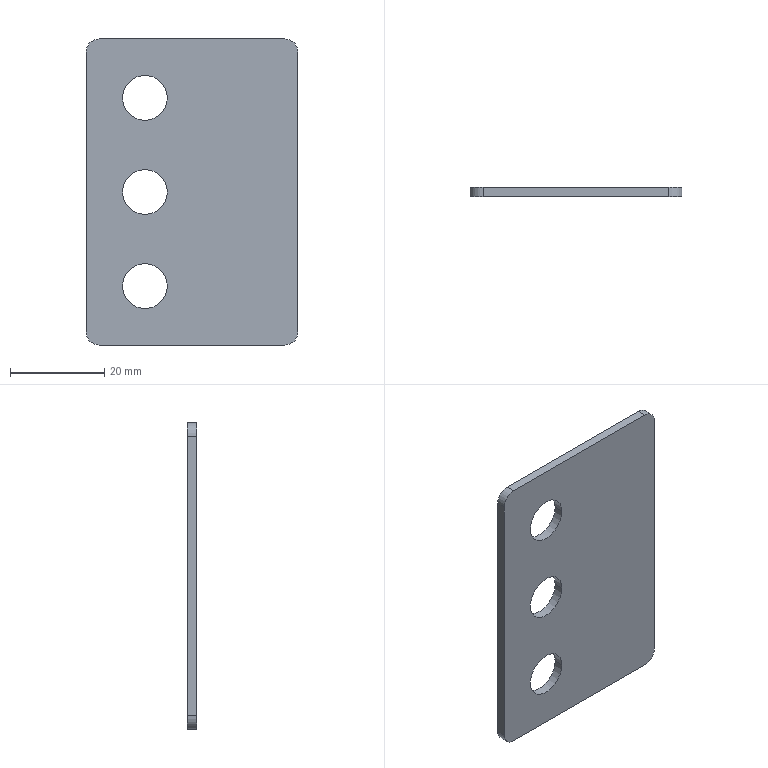Component | SolidWorks | HighVoltageMountingPlateAssembly-1_HighVoltageOutletCabinetMountingPlateSideBaffles-1 | 1 solid | 16 faces | box 45 x 2 x 65 mm | volume 5411 mm3 | cylinder 10 | plane 6 | commonest cylinder face diameters 9.5 x6 5.6 x4 | material Plain Carbon Steel
STEP:
#1=COLOUR_RGB('',0.7922,0.8196,0.9333);
#2=FILL_AREA_STYLE_COLOUR('',#1);
#3=FILL_AREA_STYLE('',(#2));
#4=SURFACE_STYLE_FILL_AREA(#3);
#5=SURFACE_SIDE_STYLE('',(#4));
#6=SURFACE_STYLE_USAGE(.BOTH.,#5);
#7=PRESENTATION_STYLE_ASSIGNMENT((#6));
#8=CARTESIAN_POINT('',(-68.137,3.52,85.837));
#9=VERTEX_POINT('',#8);
#10=CARTESIAN_POINT('',(-68.511,3.52,85.837));
#11=VERTEX_POINT('',#10);
#12=CARTESIAN_POINT('',(-68.324,3.52,85.837));
#13=DIRECTION('',(-0.,1.,-0.));
#14=DIRECTION('',(-1.,0.,0.));
#15=AXIS2_PLACEMENT_3D('',#12,#13,#14);
#16=CIRCLE('',#15,0.187);
#17=EDGE_CURVE('',#9,#11,#16,.T.);
#18=ORIENTED_EDGE('',*,*,#17,.F.);
#19=CARTESIAN_POINT('',(-68.137,3.599,85.837));
#20=VERTEX_POINT('',#19);
#21=CARTESIAN_POINT('',(-68.137,3.52,85.837));
#22=DIRECTION('',(-0.,1.,-0.));
#23=VECTOR('',#22,39.37);
#24=LINE('',#21,#23);
#25=EDGE_CURVE('',#9,#20,#24,.T.);
#26=ORIENTED_EDGE('',*,*,#25,.T.);
#27=CARTESIAN_POINT('',(-68.511,3.599,85.837));
#28=VERTEX_POINT('',#27);
#29=CARTESIAN_POINT('',(-68.324,3.599,85.837));
#30=DIRECTION('',(-0.,1.,-0.));
#31=DIRECTION('',(-1.,0.,0.));
#32=AXIS2_PLACEMENT_3D('',#29,#30,#31);
#33=CIRCLE('',#32,0.187);
#34=EDGE_CURVE('',#20,#28,#33,.T.);
#35=ORIENTED_EDGE('',*,*,#34,.T.);
#36=CARTESIAN_POINT('',(-68.511,3.52,85.837));
#37=DIRECTION('',(-0.,1.,-0.));
#38=VECTOR('',#37,39.37);
#39=LINE('',#36,#38);
#40=EDGE_CURVE('',#11,#28,#39,.T.);
#41=ORIENTED_EDGE('',*,*,#40,.F.);
#42=EDGE_LOOP('',(#18,#26,#35,#41));
#43=FACE_OUTER_BOUND('',#42,.T.);
#44=CARTESIAN_POINT('',(-68.324,3.52,85.837));
#45=DIRECTION('',(-0.,1.,-0.));
#46=DIRECTION('',(-1.,0.,0.));
#47=AXIS2_PLACEMENT_3D('',#44,#45,#46);
#48=CYLINDRICAL_SURFACE('',#47,0.187);
#49=ADVANCED_FACE('',(#43),#48,.F.);
#50=CARTESIAN_POINT('',(-68.137,3.52,85.05));
#51=VERTEX_POINT('',#50);
#52=CARTESIAN_POINT('',(-68.511,3.52,85.05));
#53=VERTEX_POINT('',#52);
#54=CARTESIAN_POINT('',(-68.324,3.52,85.05));
#55=DIRECTION('',(-0.,1.,-0.));
#56=DIRECTION('',(-1.,0.,0.));
#57=AXIS2_PLACEMENT_3D('',#54,#55,#56);
#58=CIRCLE('',#57,0.187);
#59=EDGE_CURVE('',#51,#53,#58,.T.);
#60=ORIENTED_EDGE('',*,*,#59,.F.);
#61=CARTESIAN_POINT('',(-68.137,3.599,85.05));
#62=VERTEX_POINT('',#61);
#63=CARTESIAN_POINT('',(-68.137,3.52,85.05));
#64=DIRECTION('',(-0.,1.,-0.));
#65=VECTOR('',#64,39.37);
#66=LINE('',#63,#65);
#67=EDGE_CURVE('',#51,#62,#66,.T.);
#68=ORIENTED_EDGE('',*,*,#67,.T.);
#69=CARTESIAN_POINT('',(-68.511,3.599,85.05));
#70=VERTEX_POINT('',#69);
#71=CARTESIAN_POINT('',(-68.324,3.599,85.05));
#72=DIRECTION('',(-0.,1.,-0.));
#73=DIRECTION('',(-1.,0.,0.));
#74=AXIS2_PLACEMENT_3D('',#71,#72,#73);
#75=CIRCLE('',#74,0.187);
#76=EDGE_CURVE('',#62,#70,#75,.T.);
#77=ORIENTED_EDGE('',*,*,#76,.T.);
#78=CARTESIAN_POINT('',(-68.511,3.52,85.05));
#79=DIRECTION('',(-0.,1.,-0.));
#80=VECTOR('',#79,39.37);
#81=LINE('',#78,#80);
#82=EDGE_CURVE('',#53,#70,#81,.T.);
#83=ORIENTED_EDGE('',*,*,#82,.F.);
#84=EDGE_LOOP('',(#60,#68,#77,#83));
#85=FACE_OUTER_BOUND('',#84,.T.);
#86=CARTESIAN_POINT('',(-68.324,3.52,85.05));
#87=DIRECTION('',(-0.,1.,-0.));
#88=DIRECTION('',(-1.,0.,0.));
#89=AXIS2_PLACEMENT_3D('',#86,#87,#88);
#90=CYLINDRICAL_SURFACE('',#89,0.187);
#91=ADVANCED_FACE('',(#85),#90,.F.);
#92=CARTESIAN_POINT('',(-68.137,3.52,86.625));
#93=VERTEX_POINT('',#92);
#94=CARTESIAN_POINT('',(-68.511,3.52,86.625));
#95=VERTEX_POINT('',#94);
#96=CARTESIAN_POINT('',(-68.324,3.52,86.625));
#97=DIRECTION('',(-0.,1.,-0.));
#98=DIRECTION('',(-1.,0.,0.));
#99=AXIS2_PLACEMENT_3D('',#96,#97,#98);
#100=CIRCLE('',#99,0.187);
#101=EDGE_CURVE('',#93,#95,#100,.T.);
#102=ORIENTED_EDGE('',*,*,#101,.F.);
#103=CARTESIAN_POINT('',(-68.137,3.599,86.625));
#104=VERTEX_POINT('',#103);
#105=CARTESIAN_POINT('',(-68.137,3.52,86.625));
#106=DIRECTION('',(-0.,1.,-0.));
#107=VECTOR('',#106,39.37);
#108=LINE('',#105,#107);
#109=EDGE_CURVE('',#93,#104,#108,.T.);
#110=ORIENTED_EDGE('',*,*,#109,.T.);
#111=CARTESIAN_POINT('',(-68.511,3.599,86.625));
#112=VERTEX_POINT('',#111);
#113=CARTESIAN_POINT('',(-68.324,3.599,86.625));
#114=DIRECTION('',(-0.,1.,-0.));
#115=DIRECTION('',(-1.,0.,0.));
#116=AXIS2_PLACEMENT_3D('',#113,#114,#115);
#117=CIRCLE('',#116,0.187);
#118=EDGE_CURVE('',#104,#112,#117,.T.);
#119=ORIENTED_EDGE('',*,*,#118,.T.);
#120=CARTESIAN_POINT('',(-68.511,3.52,86.625));
#121=DIRECTION('',(-0.,1.,-0.));
#122=VECTOR('',#121,39.37);
#123=LINE('',#120,#122);
#124=EDGE_CURVE('',#95,#112,#123,.T.);
#125=ORIENTED_EDGE('',*,*,#124,.F.);
#126=EDGE_LOOP('',(#102,#110,#119,#125));
#127=FACE_OUTER_BOUND('',#126,.T.);
#128=CARTESIAN_POINT('',(-68.324,3.52,86.625));
#129=DIRECTION('',(-0.,1.,-0.));
#130=DIRECTION('',(-1.,0.,0.));
#131=AXIS2_PLACEMENT_3D('',#128,#129,#130);
#132=CYLINDRICAL_SURFACE('',#131,0.187);
#133=ADVANCED_FACE('',(#127),#132,.F.);
#134=CARTESIAN_POINT('',(-67.045,3.52,87.007));
#135=VERTEX_POINT('',#134);
#136=CARTESIAN_POINT('',(-67.045,3.52,84.668));
#137=VERTEX_POINT('',#136);
#138=CARTESIAN_POINT('',(-67.045,3.52,84.558));
#139=DIRECTION('',(-0.,0.,-1.));
#140=VECTOR('',#139,39.37);
#141=LINE('',#138,#140);
#142=EDGE_CURVE('',#135,#137,#141,.T.);
#143=ORIENTED_EDGE('',*,*,#142,.T.);
#144=CARTESIAN_POINT('',(-67.045,3.599,84.668));
#145=VERTEX_POINT('',#144);
#146=CARTESIAN_POINT('',(-67.045,3.52,84.668));
#147=DIRECTION('',(-0.,1.,-0.));
#148=VECTOR('',#147,39.37);
#149=LINE('',#146,#148);
#150=EDGE_CURVE('',#137,#145,#149,.T.);
#151=ORIENTED_EDGE('',*,*,#150,.T.);
#152=CARTESIAN_POINT('',(-67.045,3.599,87.007));
#153=VERTEX_POINT('',#152);
#154=CARTESIAN_POINT('',(-67.045,3.599,84.558));
#155=DIRECTION('',(-0.,0.,-1.));
#156=VECTOR('',#155,39.37);
#157=LINE('',#154,#156);
#158=EDGE_CURVE('',#153,#145,#157,.T.);
#159=ORIENTED_EDGE('',*,*,#158,.F.);
#160=CARTESIAN_POINT('',(-67.045,3.52,87.007));
#161=DIRECTION('',(0.,-1.,0.));
#162=VECTOR('',#161,39.37);
#163=LINE('',#160,#162);
#164=EDGE_CURVE('',#153,#135,#163,.T.);
#165=ORIENTED_EDGE('',*,*,#164,.T.);
#166=EDGE_LOOP('',(#143,#151,#159,#165));
#167=FACE_OUTER_BOUND('',#166,.T.);
#168=CARTESIAN_POINT('',(-67.045,3.52,84.558));
#169=DIRECTION('',(1.,0.,0.));
#170=DIRECTION('',(-0.,1.,-0.));
#171=AXIS2_PLACEMENT_3D('',#168,#169,#170);
#172=PLANE('',#171);
#173=ADVANCED_FACE('',(#167),#172,.T.);
#174=CARTESIAN_POINT('',(-68.706,3.599,87.117));
#175=VERTEX_POINT('',#174);
#176=CARTESIAN_POINT('',(-67.155,3.599,87.117));
#177=VERTEX_POINT('',#176);
#178=CARTESIAN_POINT('',(-67.045,3.599,87.117));
#179=DIRECTION('',(1.,-0.,0.));
#180=VECTOR('',#179,39.37);
#181=LINE('',#178,#180);
#182=EDGE_CURVE('',#175,#177,#181,.T.);
#183=ORIENTED_EDGE('',*,*,#182,.F.);
#184=CARTESIAN_POINT('',(-68.706,3.52,87.117));
#185=VERTEX_POINT('',#184);
#186=CARTESIAN_POINT('',(-68.706,3.52,87.117));
#187=DIRECTION('',(0.,-1.,0.));
#188=VECTOR('',#187,39.37);
#189=LINE('',#186,#188);
#190=EDGE_CURVE('',#175,#185,#189,.T.);
#191=ORIENTED_EDGE('',*,*,#190,.T.);
#192=CARTESIAN_POINT('',(-67.155,3.52,87.117));
#193=VERTEX_POINT('',#192);
#194=CARTESIAN_POINT('',(-67.045,3.52,87.117));
#195=DIRECTION('',(1.,-0.,0.));
#196=VECTOR('',#195,39.37);
#197=LINE('',#194,#196);
#198=EDGE_CURVE('',#185,#193,#197,.T.);
#199=ORIENTED_EDGE('',*,*,#198,.T.);
#200=CARTESIAN_POINT('',(-67.155,3.52,87.117));
#201=DIRECTION('',(-0.,1.,-0.));
#202=VECTOR('',#201,39.37);
#203=LINE('',#200,#202);
#204=EDGE_CURVE('',#193,#177,#203,.T.);
#205=ORIENTED_EDGE('',*,*,#204,.T.);
#206=EDGE_LOOP('',(#183,#191,#199,#205));
#207=FACE_OUTER_BOUND('',#206,.T.);
#208=CARTESIAN_POINT('',(-67.045,3.52,87.117));
#209=DIRECTION('',(0.,0.,1.));
#210=DIRECTION('',(-0.,1.,-0.));
#211=AXIS2_PLACEMENT_3D('',#208,#209,#210);
#212=PLANE('',#211);
#213=ADVANCED_FACE('',(#207),#212,.T.);
#214=CARTESIAN_POINT('',(-68.816,3.599,84.668));
#215=VERTEX_POINT('',#214);
#216=CARTESIAN_POINT('',(-68.816,3.599,87.007));
#217=VERTEX_POINT('',#216);
#218=CARTESIAN_POINT('',(-68.816,3.599,84.558));
#219=DIRECTION('',(0.,-0.,1.));
#220=VECTOR('',#219,39.37);
#221=LINE('',#218,#220);
#222=EDGE_CURVE('',#215,#217,#221,.T.);
#223=ORIENTED_EDGE('',*,*,#222,.F.);
#224=CARTESIAN_POINT('',(-68.816,3.52,84.668));
#225=VERTEX_POINT('',#224);
#226=CARTESIAN_POINT('',(-68.816,3.52,84.668));
#227=DIRECTION('',(0.,-1.,0.));
#228=VECTOR('',#227,39.37);
#229=LINE('',#226,#228);
#230=EDGE_CURVE('',#215,#225,#229,.T.);
#231=ORIENTED_EDGE('',*,*,#230,.T.);
#232=CARTESIAN_POINT('',(-68.816,3.52,87.007));
#233=VERTEX_POINT('',#232);
#234=CARTESIAN_POINT('',(-68.816,3.52,84.558));
#235=DIRECTION('',(0.,-0.,1.));
#236=VECTOR('',#235,39.37);
#237=LINE('',#234,#236);
#238=EDGE_CURVE('',#225,#233,#237,.T.);
#239=ORIENTED_EDGE('',*,*,#238,.T.);
#240=CARTESIAN_POINT('',(-68.816,3.52,87.007));
#241=DIRECTION('',(-0.,1.,-0.));
#242=VECTOR('',#241,39.37);
#243=LINE('',#240,#242);
#244=EDGE_CURVE('',#233,#217,#243,.T.);
#245=ORIENTED_EDGE('',*,*,#244,.T.);
#246=EDGE_LOOP('',(#223,#231,#239,#245));
#247=FACE_OUTER_BOUND('',#246,.T.);
#248=CARTESIAN_POINT('',(-68.816,3.52,84.558));
#249=DIRECTION('',(-1.,-0.,-0.));
#250=DIRECTION('',(0.,-1.,0.));
#251=AXIS2_PLACEMENT_3D('',#248,#249,#250);
#252=PLANE('',#251);
#253=ADVANCED_FACE('',(#247),#252,.T.);
#254=CARTESIAN_POINT('',(-67.155,3.599,84.558));
#255=VERTEX_POINT('',#254);
#256=CARTESIAN_POINT('',(-68.706,3.599,84.558));
#257=VERTEX_POINT('',#256);
#258=CARTESIAN_POINT('',(-67.045,3.599,84.558));
#259=DIRECTION('',(-1.,0.,-0.));
#260=VECTOR('',#259,39.37);
#261=LINE('',#258,#260);
#262=EDGE_CURVE('',#255,#257,#261,.T.);
#263=ORIENTED_EDGE('',*,*,#262,.F.);
#264=CARTESIAN_POINT('',(-67.155,3.52,84.558));
#265=VERTEX_POINT('',#264);
#266=CARTESIAN_POINT('',(-67.155,3.52,84.558));
#267=DIRECTION('',(0.,-1.,0.));
#268=VECTOR('',#267,39.37);
#269=LINE('',#266,#268);
#270=EDGE_CURVE('',#255,#265,#269,.T.);
#271=ORIENTED_EDGE('',*,*,#270,.T.);
#272=CARTESIAN_POINT('',(-68.706,3.52,84.558));
#273=VERTEX_POINT('',#272);
#274=CARTESIAN_POINT('',(-67.045,3.52,84.558));
#275=DIRECTION('',(-1.,0.,-0.));
#276=VECTOR('',#275,39.37);
#277=LINE('',#274,#276);
#278=EDGE_CURVE('',#265,#273,#277,.T.);
#279=ORIENTED_EDGE('',*,*,#278,.T.);
#280=CARTESIAN_POINT('',(-68.706,3.52,84.558));
#281=DIRECTION('',(-0.,1.,-0.));
#282=VECTOR('',#281,39.37);
#283=LINE('',#280,#282);
#284=EDGE_CURVE('',#273,#257,#283,.T.);
#285=ORIENTED_EDGE('',*,*,#284,.T.);
#286=EDGE_LOOP('',(#263,#271,#279,#285));
#287=FACE_OUTER_BOUND('',#286,.T.);
#288=CARTESIAN_POINT('',(-67.045,3.52,84.558));
#289=DIRECTION('',(-0.,-0.,-1.));
#290=DIRECTION('',(0.,-1.,0.));
#291=AXIS2_PLACEMENT_3D('',#288,#289,#290);
#292=PLANE('',#291);
#293=ADVANCED_FACE('',(#287),#292,.T.);
#294=CARTESIAN_POINT('',(-68.324,3.52,85.837));
#295=DIRECTION('',(-0.,1.,-0.));
#296=DIRECTION('',(-1.,0.,0.));
#297=AXIS2_PLACEMENT_3D('',#294,#295,#296);
#298=CIRCLE('',#297,0.187);
#299=EDGE_CURVE('',#11,#9,#298,.T.);
#300=ORIENTED_EDGE('',*,*,#299,.T.);
#301=ORIENTED_EDGE('',*,*,#17,.T.);
#302=EDGE_LOOP('',(#300,#301));
#303=FACE_BOUND('',#302,.T.);
#304=CARTESIAN_POINT('',(-68.324,3.52,85.05));
#305=DIRECTION('',(-0.,1.,-0.));
#306=DIRECTION('',(-1.,0.,0.));
#307=AXIS2_PLACEMENT_3D('',#304,#305,#306);
#308=CIRCLE('',#307,0.187);
#309=EDGE_CURVE('',#53,#51,#308,.T.);
#310=ORIENTED_EDGE('',*,*,#309,.T.);
#311=ORIENTED_EDGE('',*,*,#59,.T.);
#312=EDGE_LOOP('',(#310,#311));
#313=FACE_BOUND('',#312,.T.);
#314=CARTESIAN_POINT('',(-68.324,3.52,86.625));
#315=DIRECTION('',(-0.,1.,-0.));
#316=DIRECTION('',(-1.,0.,0.));
#317=AXIS2_PLACEMENT_3D('',#314,#315,#316);
#318=CIRCLE('',#317,0.187);
#319=EDGE_CURVE('',#95,#93,#318,.T.);
#320=ORIENTED_EDGE('',*,*,#319,.T.);
#321=ORIENTED_EDGE('',*,*,#101,.T.);
#322=EDGE_LOOP('',(#320,#321));
#323=FACE_BOUND('',#322,.T.);
#324=ORIENTED_EDGE('',*,*,#278,.F.);
#325=CARTESIAN_POINT('',(-67.155,3.52,84.668));
#326=DIRECTION('',(0.,-1.,0.));
#327=DIRECTION('',(1.,0.,0.));
#328=AXIS2_PLACEMENT_3D('',#325,#326,#327);
#329=CIRCLE('',#328,0.1102);
#330=EDGE_CURVE('',#265,#137,#329,.T.);
#331=ORIENTED_EDGE('',*,*,#330,.T.);
#332=ORIENTED_EDGE('',*,*,#142,.F.);
#333=CARTESIAN_POINT('',(-67.155,3.52,87.007));
#334=DIRECTION('',(0.,-1.,0.));
#335=DIRECTION('',(1.,0.,0.));
#336=AXIS2_PLACEMENT_3D('',#333,#334,#335);
#337=CIRCLE('',#336,0.1102);
#338=EDGE_CURVE('',#135,#193,#337,.T.);
#339=ORIENTED_EDGE('',*,*,#338,.T.);
#340=ORIENTED_EDGE('',*,*,#198,.F.);
#341=CARTESIAN_POINT('',(-68.706,3.52,87.007));
#342=DIRECTION('',(0.,-1.,0.));
#343=DIRECTION('',(1.,0.,0.));
#344=AXIS2_PLACEMENT_3D('',#341,#342,#343);
#345=CIRCLE('',#344,0.1102);
#346=EDGE_CURVE('',#185,#233,#345,.T.);
#347=ORIENTED_EDGE('',*,*,#346,.T.);
#348=ORIENTED_EDGE('',*,*,#238,.F.);
#349=CARTESIAN_POINT('',(-68.706,3.52,84.668));
#350=DIRECTION('',(0.,-1.,0.));
#351=DIRECTION('',(1.,0.,0.));
#352=AXIS2_PLACEMENT_3D('',#349,#350,#351);
#353=CIRCLE('',#352,0.1102);
#354=EDGE_CURVE('',#225,#273,#353,.T.);
#355=ORIENTED_EDGE('',*,*,#354,.T.);
#356=EDGE_LOOP('',(#324,#331,#332,#339,#340,#347,#348,#355));
#357=FACE_OUTER_BOUND('',#356,.T.);
#358=CARTESIAN_POINT('',(-67.045,3.52,84.558));
#359=DIRECTION('',(-0.,-1.,0.));
#360=DIRECTION('',(1.,-0.,0.));
#361=AXIS2_PLACEMENT_3D('',#358,#359,#360);
#362=PLANE('',#361);
#363=ADVANCED_FACE('',(#303,#313,#323,#357),#362,.T.);
#364=CARTESIAN_POINT('',(-68.324,3.599,85.837));
#365=DIRECTION('',(-0.,1.,-0.));
#366=DIRECTION('',(-1.,0.,0.));
#367=AXIS2_PLACEMENT_3D('',#364,#365,#366);
#368=CIRCLE('',#367,0.187);
#369=EDGE_CURVE('',#28,#20,#368,.T.);
#370=ORIENTED_EDGE('',*,*,#369,.F.);
#371=ORIENTED_EDGE('',*,*,#34,.F.);
#372=EDGE_LOOP('',(#370,#371));
#373=FACE_BOUND('',#372,.T.);
#374=CARTESIAN_POINT('',(-68.324,3.599,85.05));
#375=DIRECTION('',(-0.,1.,-0.));
#376=DIRECTION('',(-1.,0.,0.));
#377=AXIS2_PLACEMENT_3D('',#374,#375,#376);
#378=CIRCLE('',#377,0.187);
#379=EDGE_CURVE('',#70,#62,#378,.T.);
#380=ORIENTED_EDGE('',*,*,#379,.F.);
#381=ORIENTED_EDGE('',*,*,#76,.F.);
#382=EDGE_LOOP('',(#380,#381));
#383=FACE_BOUND('',#382,.T.);
#384=CARTESIAN_POINT('',(-68.324,3.599,86.625));
#385=DIRECTION('',(-0.,1.,-0.));
#386=DIRECTION('',(-1.,0.,0.));
#387=AXIS2_PLACEMENT_3D('',#384,#385,#386);
#388=CIRCLE('',#387,0.187);
#389=EDGE_CURVE('',#112,#104,#388,.T.);
#390=ORIENTED_EDGE('',*,*,#389,.F.);
#391=ORIENTED_EDGE('',*,*,#118,.F.);
#392=EDGE_LOOP('',(#390,#391));
#393=FACE_BOUND('',#392,.T.);
#394=ORIENTED_EDGE('',*,*,#158,.T.);
#395=CARTESIAN_POINT('',(-67.155,3.599,84.668));
#396=DIRECTION('',(-0.,1.,-0.));
#397=DIRECTION('',(1.,0.,0.));
#398=AXIS2_PLACEMENT_3D('',#395,#396,#397);
#399=CIRCLE('',#398,0.1102);
#400=EDGE_CURVE('',#145,#255,#399,.T.);
#401=ORIENTED_EDGE('',*,*,#400,.T.);
#402=ORIENTED_EDGE('',*,*,#262,.T.);
#403=CARTESIAN_POINT('',(-68.706,3.599,84.668));
#404=DIRECTION('',(-0.,1.,-0.));
#405=DIRECTION('',(1.,0.,0.));
#406=AXIS2_PLACEMENT_3D('',#403,#404,#405);
#407=CIRCLE('',#406,0.1102);
#408=EDGE_CURVE('',#257,#215,#407,.T.);
#409=ORIENTED_EDGE('',*,*,#408,.T.);
#410=ORIENTED_EDGE('',*,*,#222,.T.);
#411=CARTESIAN_POINT('',(-68.706,3.599,87.007));
#412=DIRECTION('',(-0.,1.,-0.));
#413=DIRECTION('',(1.,0.,0.));
#414=AXIS2_PLACEMENT_3D('',#411,#412,#413);
#415=CIRCLE('',#414,0.1102);
#416=EDGE_CURVE('',#217,#175,#415,.T.);
#417=ORIENTED_EDGE('',*,*,#416,.T.);
#418=ORIENTED_EDGE('',*,*,#182,.T.);
#419=CARTESIAN_POINT('',(-67.155,3.599,87.007));
#420=DIRECTION('',(-0.,1.,-0.));
#421=DIRECTION('',(1.,0.,0.));
#422=AXIS2_PLACEMENT_3D('',#419,#420,#421);
#423=CIRCLE('',#422,0.1102);
#424=EDGE_CURVE('',#177,#153,#423,.T.);
#425=ORIENTED_EDGE('',*,*,#424,.T.);
#426=EDGE_LOOP('',(#394,#401,#402,#409,#410,#417,#418,#425));
#427=FACE_OUTER_BOUND('',#426,.T.);
#428=CARTESIAN_POINT('',(-67.045,3.599,84.558));
#429=DIRECTION('',(-0.,-1.,0.));
#430=DIRECTION('',(1.,-0.,0.));
#431=AXIS2_PLACEMENT_3D('',#428,#429,#430);
#432=PLANE('',#431);
#433=ADVANCED_FACE('',(#373,#383,#393,#427),#432,.F.);
#434=ORIENTED_EDGE('',*,*,#109,.F.);
#435=ORIENTED_EDGE('',*,*,#319,.F.);
#436=ORIENTED_EDGE('',*,*,#124,.T.);
#437=ORIENTED_EDGE('',*,*,#389,.T.);
#438=EDGE_LOOP('',(#434,#435,#436,#437));
#439=FACE_OUTER_BOUND('',#438,.T.);
#440=CARTESIAN_POINT('',(-68.324,3.52,86.625));
#441=DIRECTION('',(-0.,1.,-0.));
#442=DIRECTION('',(-1.,0.,0.));
#443=AXIS2_PLACEMENT_3D('',#440,#441,#442);
#444=CYLINDRICAL_SURFACE('',#443,0.187);
#445=ADVANCED_FACE('',(#439),#444,.F.);
#446=ORIENTED_EDGE('',*,*,#67,.F.);
#447=ORIENTED_EDGE('',*,*,#309,.F.);
#448=ORIENTED_EDGE('',*,*,#82,.T.);
#449=ORIENTED_EDGE('',*,*,#379,.T.);
#450=EDGE_LOOP('',(#446,#447,#448,#449));
#451=FACE_OUTER_BOUND('',#450,.T.);
#452=CARTESIAN_POINT('',(-68.324,3.52,85.05));
#453=DIRECTION('',(-0.,1.,-0.));
#454=DIRECTION('',(-1.,0.,0.));
#455=AXIS2_PLACEMENT_3D('',#452,#453,#454);
#456=CYLINDRICAL_SURFACE('',#455,0.187);
#457=ADVANCED_FACE('',(#451),#456,.F.);
#458=ORIENTED_EDGE('',*,*,#25,.F.);
#459=ORIENTED_EDGE('',*,*,#299,.F.);
#460=ORIENTED_EDGE('',*,*,#40,.T.);
#461=ORIENTED_EDGE('',*,*,#369,.T.);
#462=EDGE_LOOP('',(#458,#459,#460,#461));
#463=FACE_OUTER_BOUND('',#462,.T.);
#464=CARTESIAN_POINT('',(-68.324,3.52,85.837));
#465=DIRECTION('',(-0.,1.,-0.));
#466=DIRECTION('',(-1.,0.,0.));
#467=AXIS2_PLACEMENT_3D('',#464,#465,#466);
#468=CYLINDRICAL_SURFACE('',#467,0.187);
#469=ADVANCED_FACE('',(#463),#468,.F.);
#470=ORIENTED_EDGE('',*,*,#330,.F.);
#471=ORIENTED_EDGE('',*,*,#270,.F.);
#472=ORIENTED_EDGE('',*,*,#400,.F.);
#473=ORIENTED_EDGE('',*,*,#150,.F.);
#474=EDGE_LOOP('',(#470,#471,#472,#473));
#475=FACE_OUTER_BOUND('',#474,.T.);
#476=CARTESIAN_POINT('',(-67.155,3.52,84.668));
#477=DIRECTION('',(-0.,1.,-0.));
#478=DIRECTION('',(-1.,0.,0.));
#479=AXIS2_PLACEMENT_3D('',#476,#477,#478);
#480=CYLINDRICAL_SURFACE('',#479,0.1102);
#481=ADVANCED_FACE('',(#475),#480,.T.);
#482=ORIENTED_EDGE('',*,*,#354,.F.);
#483=ORIENTED_EDGE('',*,*,#230,.F.);
#484=ORIENTED_EDGE('',*,*,#408,.F.);
#485=ORIENTED_EDGE('',*,*,#284,.F.);
#486=EDGE_LOOP('',(#482,#483,#484,#485));
#487=FACE_OUTER_BOUND('',#486,.T.);
#488=CARTESIAN_POINT('',(-68.706,3.52,84.668));
#489=DIRECTION('',(-0.,1.,-0.));
#490=DIRECTION('',(-1.,0.,0.));
#491=AXIS2_PLACEMENT_3D('',#488,#489,#490);
#492=CYLINDRICAL_SURFACE('',#491,0.1102);
#493=ADVANCED_FACE('',(#487),#492,.T.);
#494=ORIENTED_EDGE('',*,*,#346,.F.);
#495=ORIENTED_EDGE('',*,*,#190,.F.);
#496=ORIENTED_EDGE('',*,*,#416,.F.);
#497=ORIENTED_EDGE('',*,*,#244,.F.);
#498=EDGE_LOOP('',(#494,#495,#496,#497));
#499=FACE_OUTER_BOUND('',#498,.T.);
#500=CARTESIAN_POINT('',(-68.706,3.52,87.007));
#501=DIRECTION('',(-0.,1.,-0.));
#502=DIRECTION('',(-1.,0.,0.));
#503=AXIS2_PLACEMENT_3D('',#500,#501,#502);
#504=CYLINDRICAL_SURFACE('',#503,0.1102);
#505=ADVANCED_FACE('',(#499),#504,.T.);
#506=ORIENTED_EDGE('',*,*,#338,.F.);
#507=ORIENTED_EDGE('',*,*,#164,.F.);
#508=ORIENTED_EDGE('',*,*,#424,.F.);
#509=ORIENTED_EDGE('',*,*,#204,.F.);
#510=EDGE_LOOP('',(#506,#507,#508,#509));
#511=FACE_OUTER_BOUND('',#510,.T.);
#512=CARTESIAN_POINT('',(-67.155,3.52,87.007));
#513=DIRECTION('',(-0.,1.,-0.));
#514=DIRECTION('',(-1.,0.,0.));
#515=AXIS2_PLACEMENT_3D('',#512,#513,#514);
#516=CYLINDRICAL_SURFACE('',#515,0.1102);
#517=ADVANCED_FACE('',(#511),#516,.T.);
#518=CLOSED_SHELL('',(#49,#91,#133,#173,#213,#253,#293,#363,#433,#445,#457,#469,#481,#493,#505,#517));
#519=MANIFOLD_SOLID_BREP('',#518);
#520=STYLED_ITEM('',(#7),#519);
#521=PRESENTATION_LAYER_ASSIGNMENT('','',(#520));
#522=CARTESIAN_POINT('',(0.,0.,0.));
#523=DIRECTION('',(0.,0.,1.));
#524=DIRECTION('',(1.,0.,0.));
#525=AXIS2_PLACEMENT_3D('',#522,#523,#524);
#526=(LENGTH_UNIT()NAMED_UNIT(*)SI_UNIT($,.METRE.));
#527=LENGTH_MEASURE_WITH_UNIT(LENGTH_MEASURE(0.0254),#526);
#528=DIMENSIONAL_EXPONENTS(1.,0.,0.,0.,0.,0.,0.);
#529=(CONVERSION_BASED_UNIT('',#527)LENGTH_UNIT()NAMED_UNIT(#528));
#530=UNCERTAINTY_MEASURE_WITH_UNIT(LENGTH_MEASURE(0.00001),#529,'','');
#531=(NAMED_UNIT(*)PLANE_ANGLE_UNIT()SI_UNIT($,.RADIAN.));
#532=(NAMED_UNIT(*)SI_UNIT($,.STERADIAN.)SOLID_ANGLE_UNIT());
#533=(GEOMETRIC_REPRESENTATION_CONTEXT(3)GLOBAL_UNCERTAINTY_ASSIGNED_CONTEXT((#530))GLOBAL_UNIT_ASSIGNED_CONTEXT((#529,#531,#532))REPRESENTATION_CONTEXT('',''));
#534=ADVANCED_BREP_SHAPE_REPRESENTATION('',(#519,#525),#533);
#535=(LENGTH_UNIT()NAMED_UNIT(*)SI_UNIT($,.METRE.));
#536=LENGTH_MEASURE_WITH_UNIT(LENGTH_MEASURE(0.0254),#535);
#537=DIMENSIONAL_EXPONENTS(1.,0.,0.,0.,0.,0.,0.);
#538=(CONVERSION_BASED_UNIT('',#536)LENGTH_UNIT()NAMED_UNIT(#537));
#539=UNCERTAINTY_MEASURE_WITH_UNIT(LENGTH_MEASURE(0.00001),#538,'','');
#540=(NAMED_UNIT(*)PLANE_ANGLE_UNIT()SI_UNIT($,.RADIAN.));
#541=(NAMED_UNIT(*)SI_UNIT($,.STERADIAN.)SOLID_ANGLE_UNIT());
#542=(GEOMETRIC_REPRESENTATION_CONTEXT(3)GLOBAL_UNCERTAINTY_ASSIGNED_CONTEXT((#539))GLOBAL_UNIT_ASSIGNED_CONTEXT((#538,#540,#541))REPRESENTATION_CONTEXT('',''));
#543=MECHANICAL_DESIGN_GEOMETRIC_PRESENTATION_REPRESENTATION('',(#520),#542);